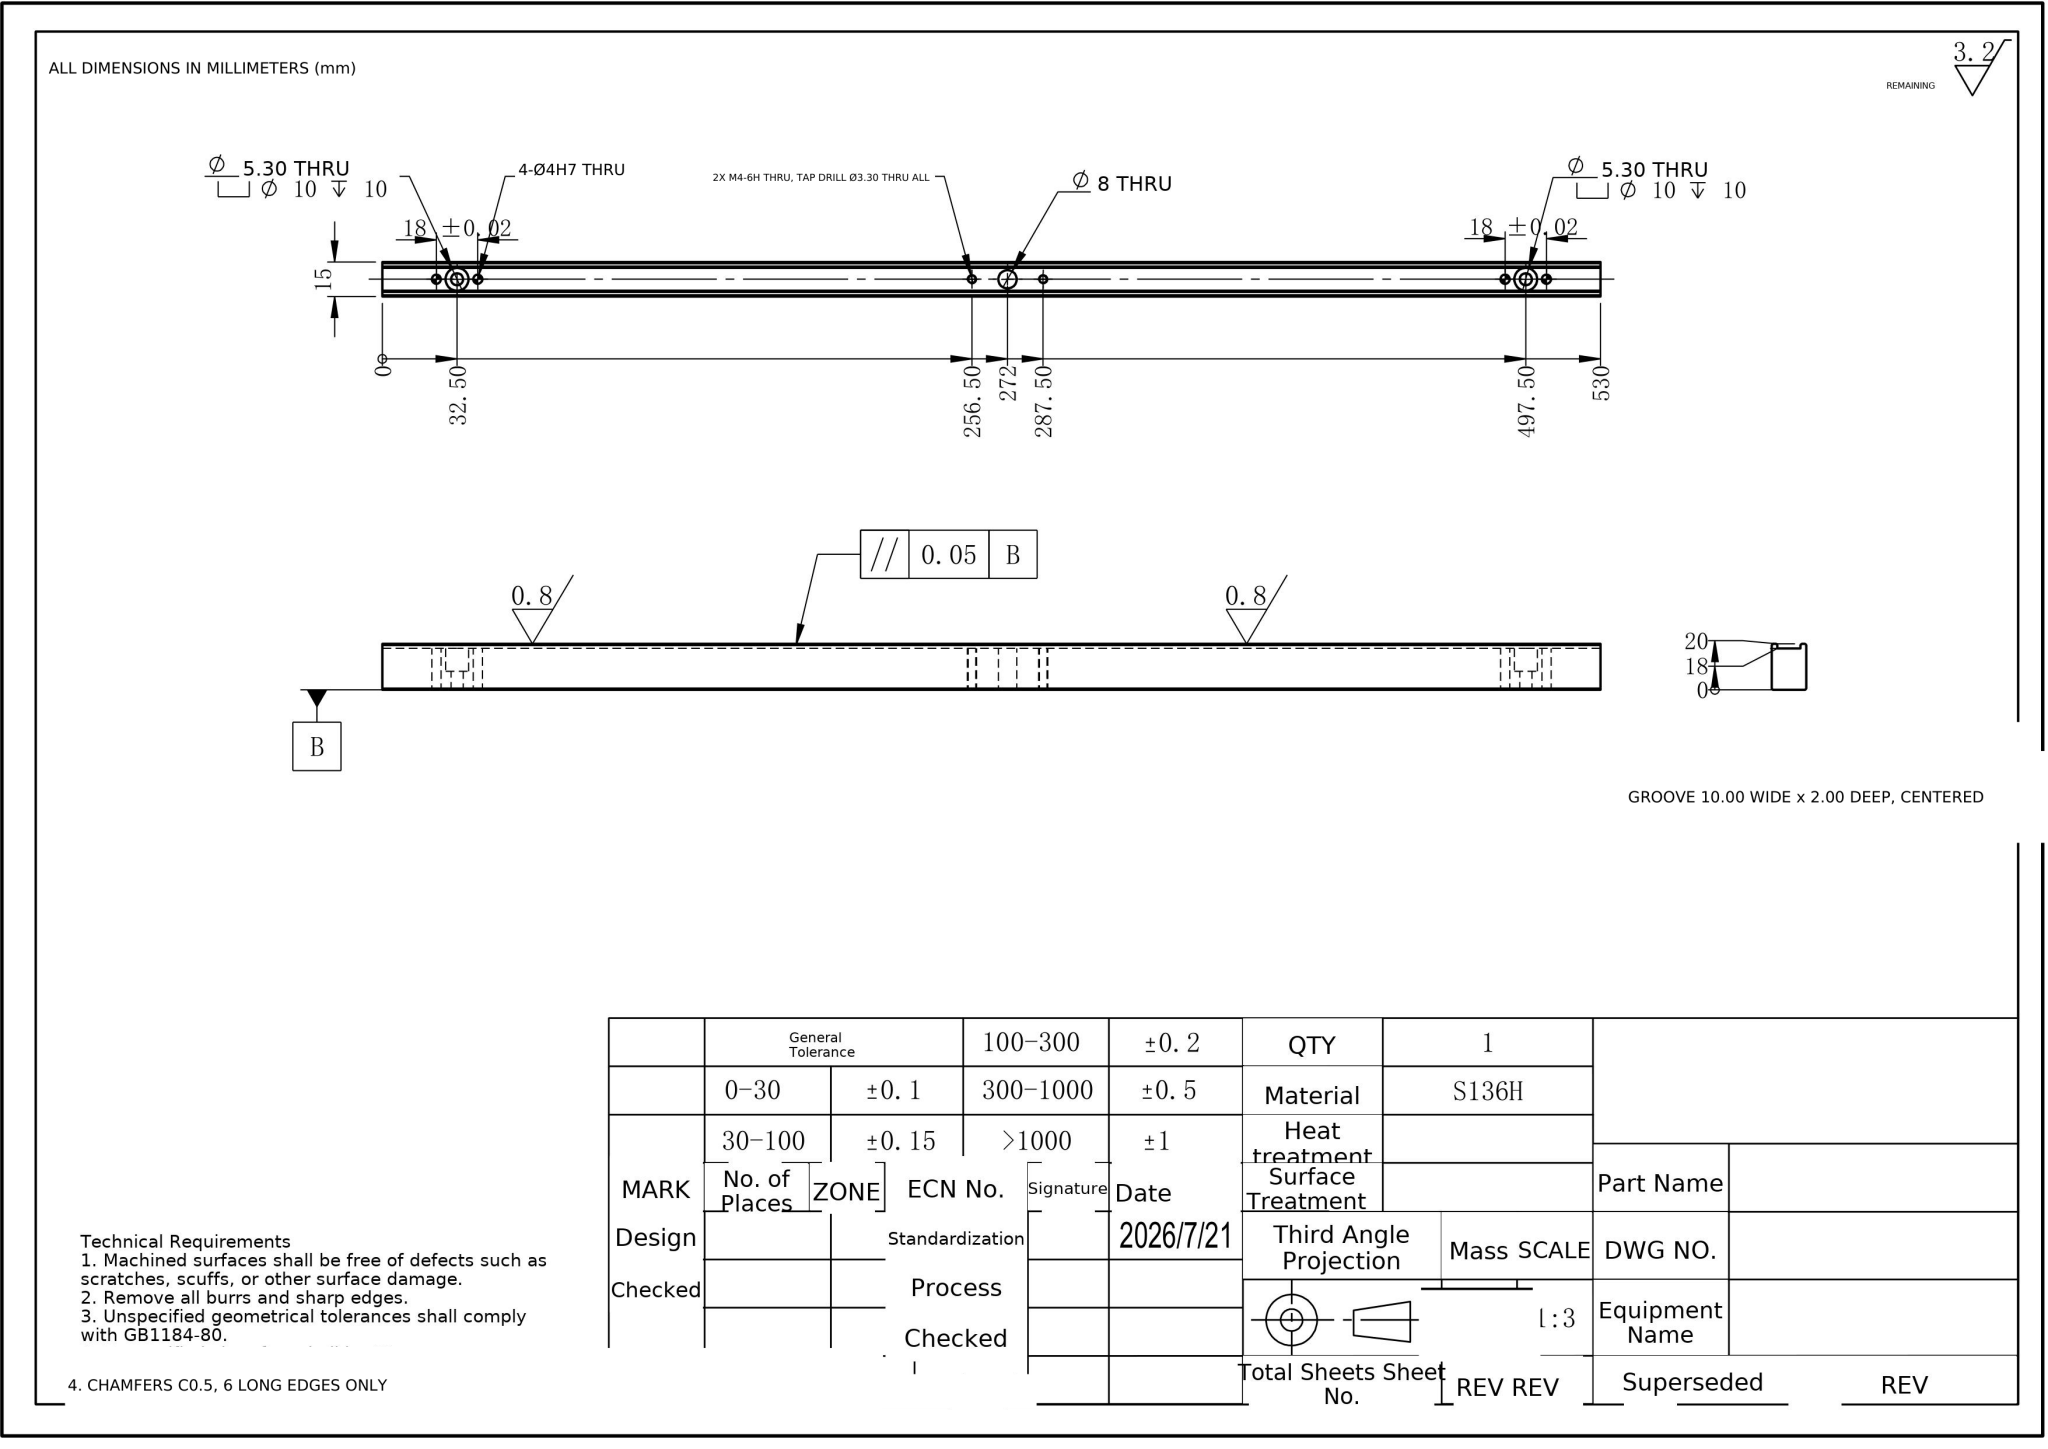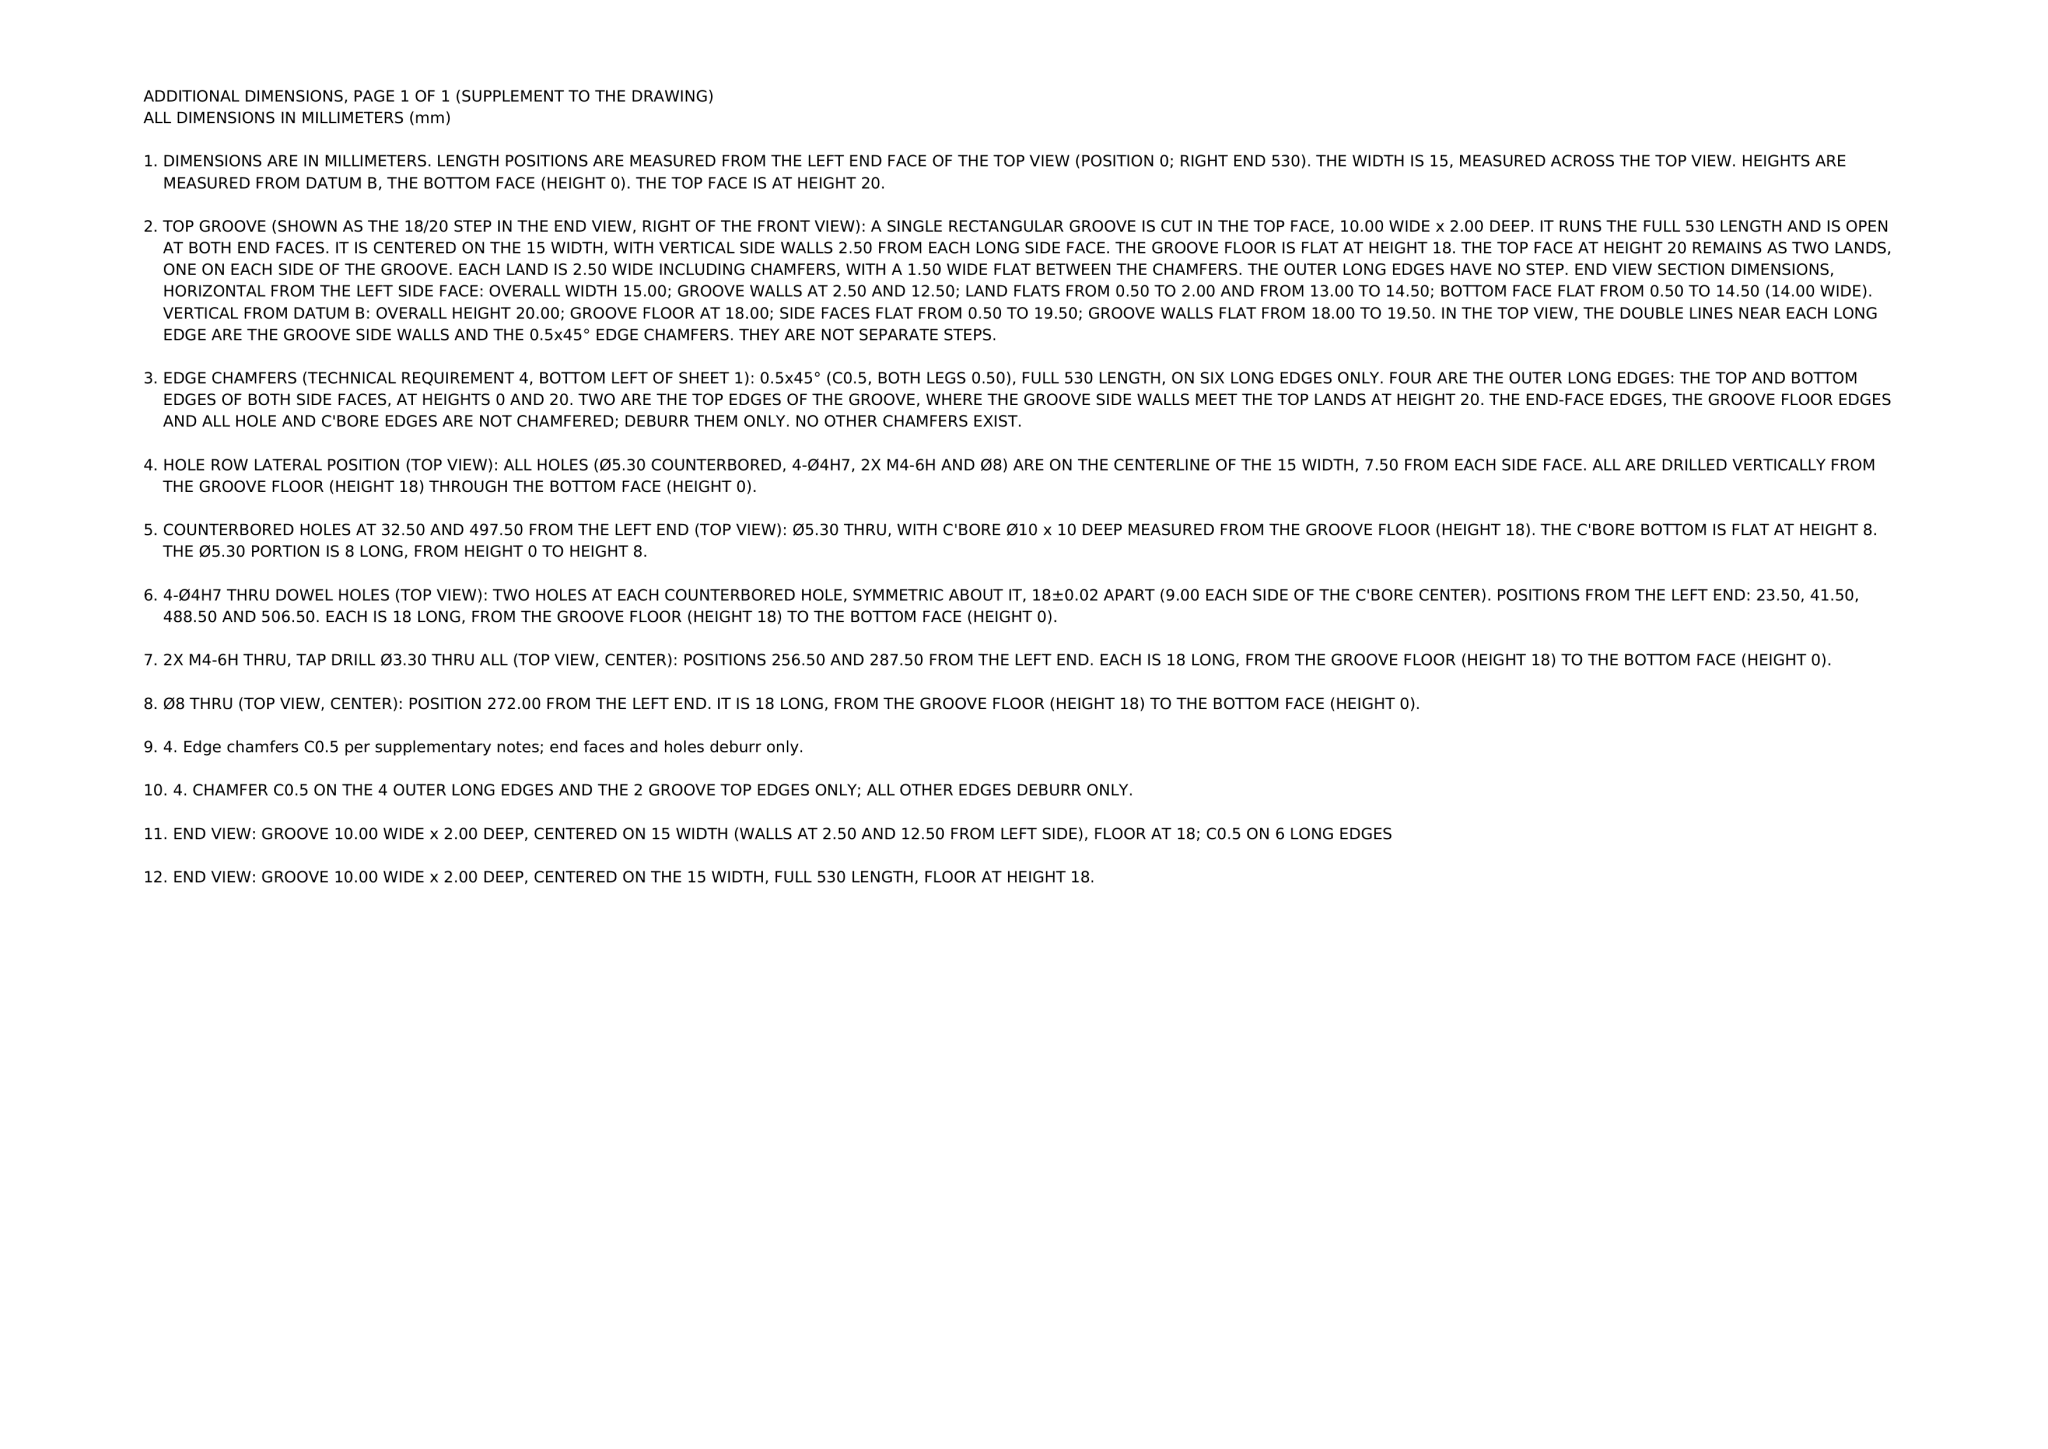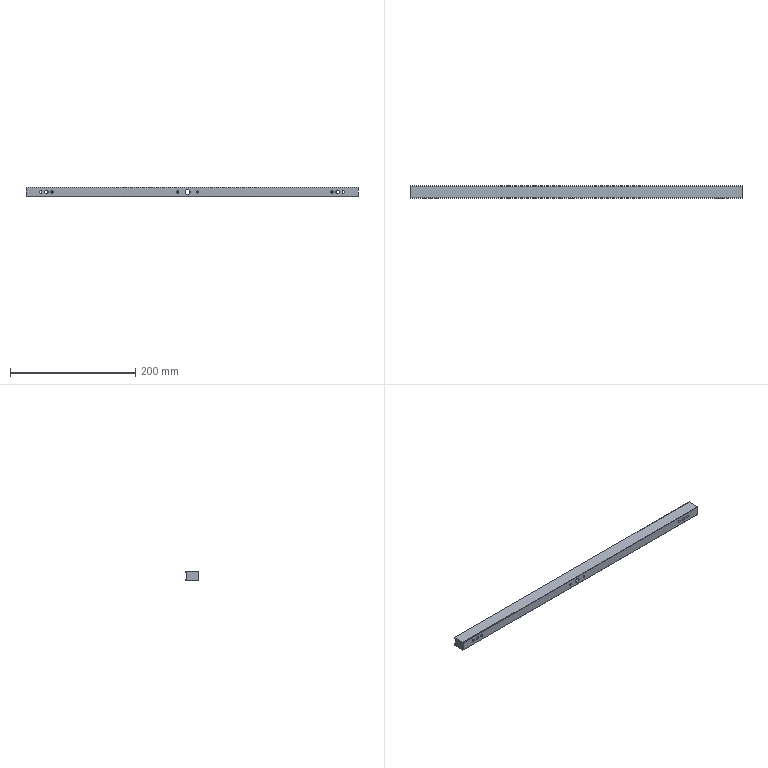Part | NX | mm | 1 solid | 42 faces | box 530 x 20 x 15 mm | volume 143961 mm3 | cylinder 22 | plane 20 | commonest cylinder face diameters 4 x8 3.3 x4 10 x4 5.3 x4 8 x2